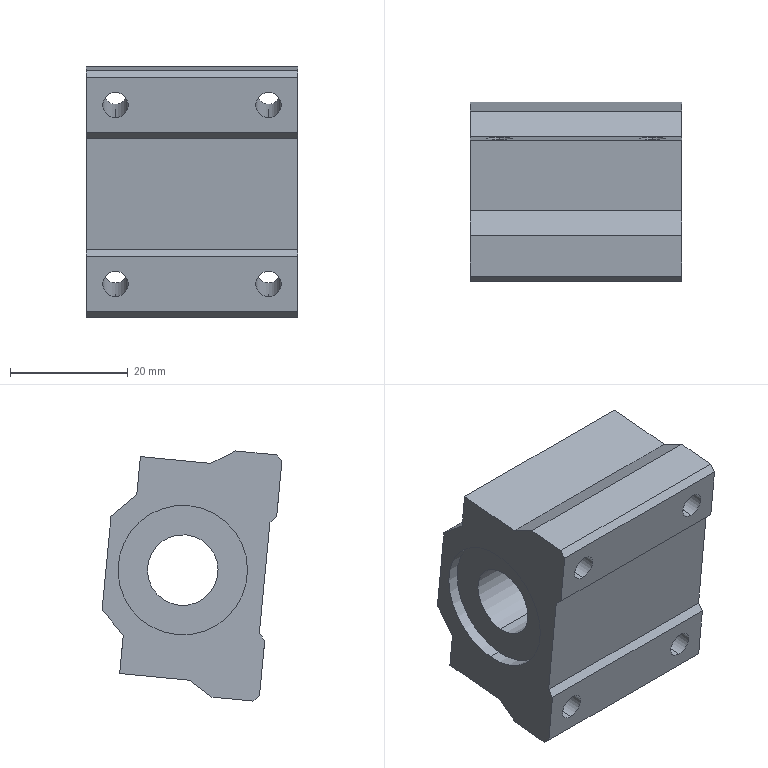Component | SolidWorks | InnerDiameter12Slider-2 | 1 solid | 36 faces | box 36 x 30.54 x 42.47 mm | volume 29327 mm3 | plane 22 | cylinder 14 | commonest cylinder face diameters 4.3 x8 22 x4 12 x2 | material Aluminum Oxide
build123d program:
from build123d import *

# Parameters (mm, degrees)
SKETCH1_R           = 6
BOSS_EXTRUDE1_DEPTH = 36
SKETCH2_R           = 11
CUT_EXTRUDE1_DEPTH  = 2
CUT_EXTRUDE2_START  = -2
SKETCH3_R           = 11
CUT_EXTRUDE2_DEPTH  = 2
SKETCH4_R           = 2.15
CUT_EXTRUDE3_DEPTH  = 51.21


with BuildPart() as part:
    # Sketch1 → Boss-Extrude1 (new body)
    with BuildSketch(Plane(origin=(0, 0, 0), x_dir=(0, 0, -1), z_dir=(1, 0, 0))):
        Polygon((-21, -7), (-18.5, -3), (-18.5, 9), (-12, 9), (-8, 13), (8, 13), (12, 9), (18.5, 9), (18.5, -3), (21, -7), (21, -13.962), (19.962, -15), (10.538, -15), (9.5, -13.962), (-9.5, -13.962), (-10.538, -15), (-19.962, -15), (-21, -13.962), align=None)
        Circle(SKETCH1_R, mode=Mode.SUBTRACT)
    extrude(amount=BOSS_EXTRUDE1_DEPTH)

    # Sketch2 → Cut-Extrude1 (cut)
    with BuildSketch(Plane(origin=(36, 0, 0), x_dir=(0, 0, -1), z_dir=(1, 0, 0))):
        Circle(SKETCH2_R)
    extrude(amount=-CUT_EXTRUDE1_DEPTH, mode=Mode.SUBTRACT)

    # Sketch3 → Cut-Extrude2 (cut)
    with BuildSketch(Plane.ZY.offset(CUT_EXTRUDE2_START)):
        with Locations(Location((0, 0, 0), (0, 0, 180))):
            Circle(SKETCH3_R)
    extrude(amount=CUT_EXTRUDE2_DEPTH, mode=Mode.SUBTRACT)

    # Sketch4 → Cut-Extrude3 (cut, through all)
    with BuildSketch(Plane.XZ.offset(15)):
        with Locations(Location((5, 15.25, 0), (0, 0, 270))):
            Circle(SKETCH4_R)
        with Locations(Location((31, 15.25, 0), (0, 0, 270))):
            Circle(SKETCH4_R)
        with Locations(Location((5, -15.25, 0), (0, 0, 270))):
            Circle(SKETCH4_R)
        with Locations(Location((31, -15.25, 0), (0, 0, 270))):
            Circle(SKETCH4_R)
    extrude(amount=-CUT_EXTRUDE3_DEPTH, mode=Mode.SUBTRACT)


solid = part.part

# Placed as in the assembly
solid = solid.moved(Location((294.062, 15.116, 349), (-174.519, 0, 180)))